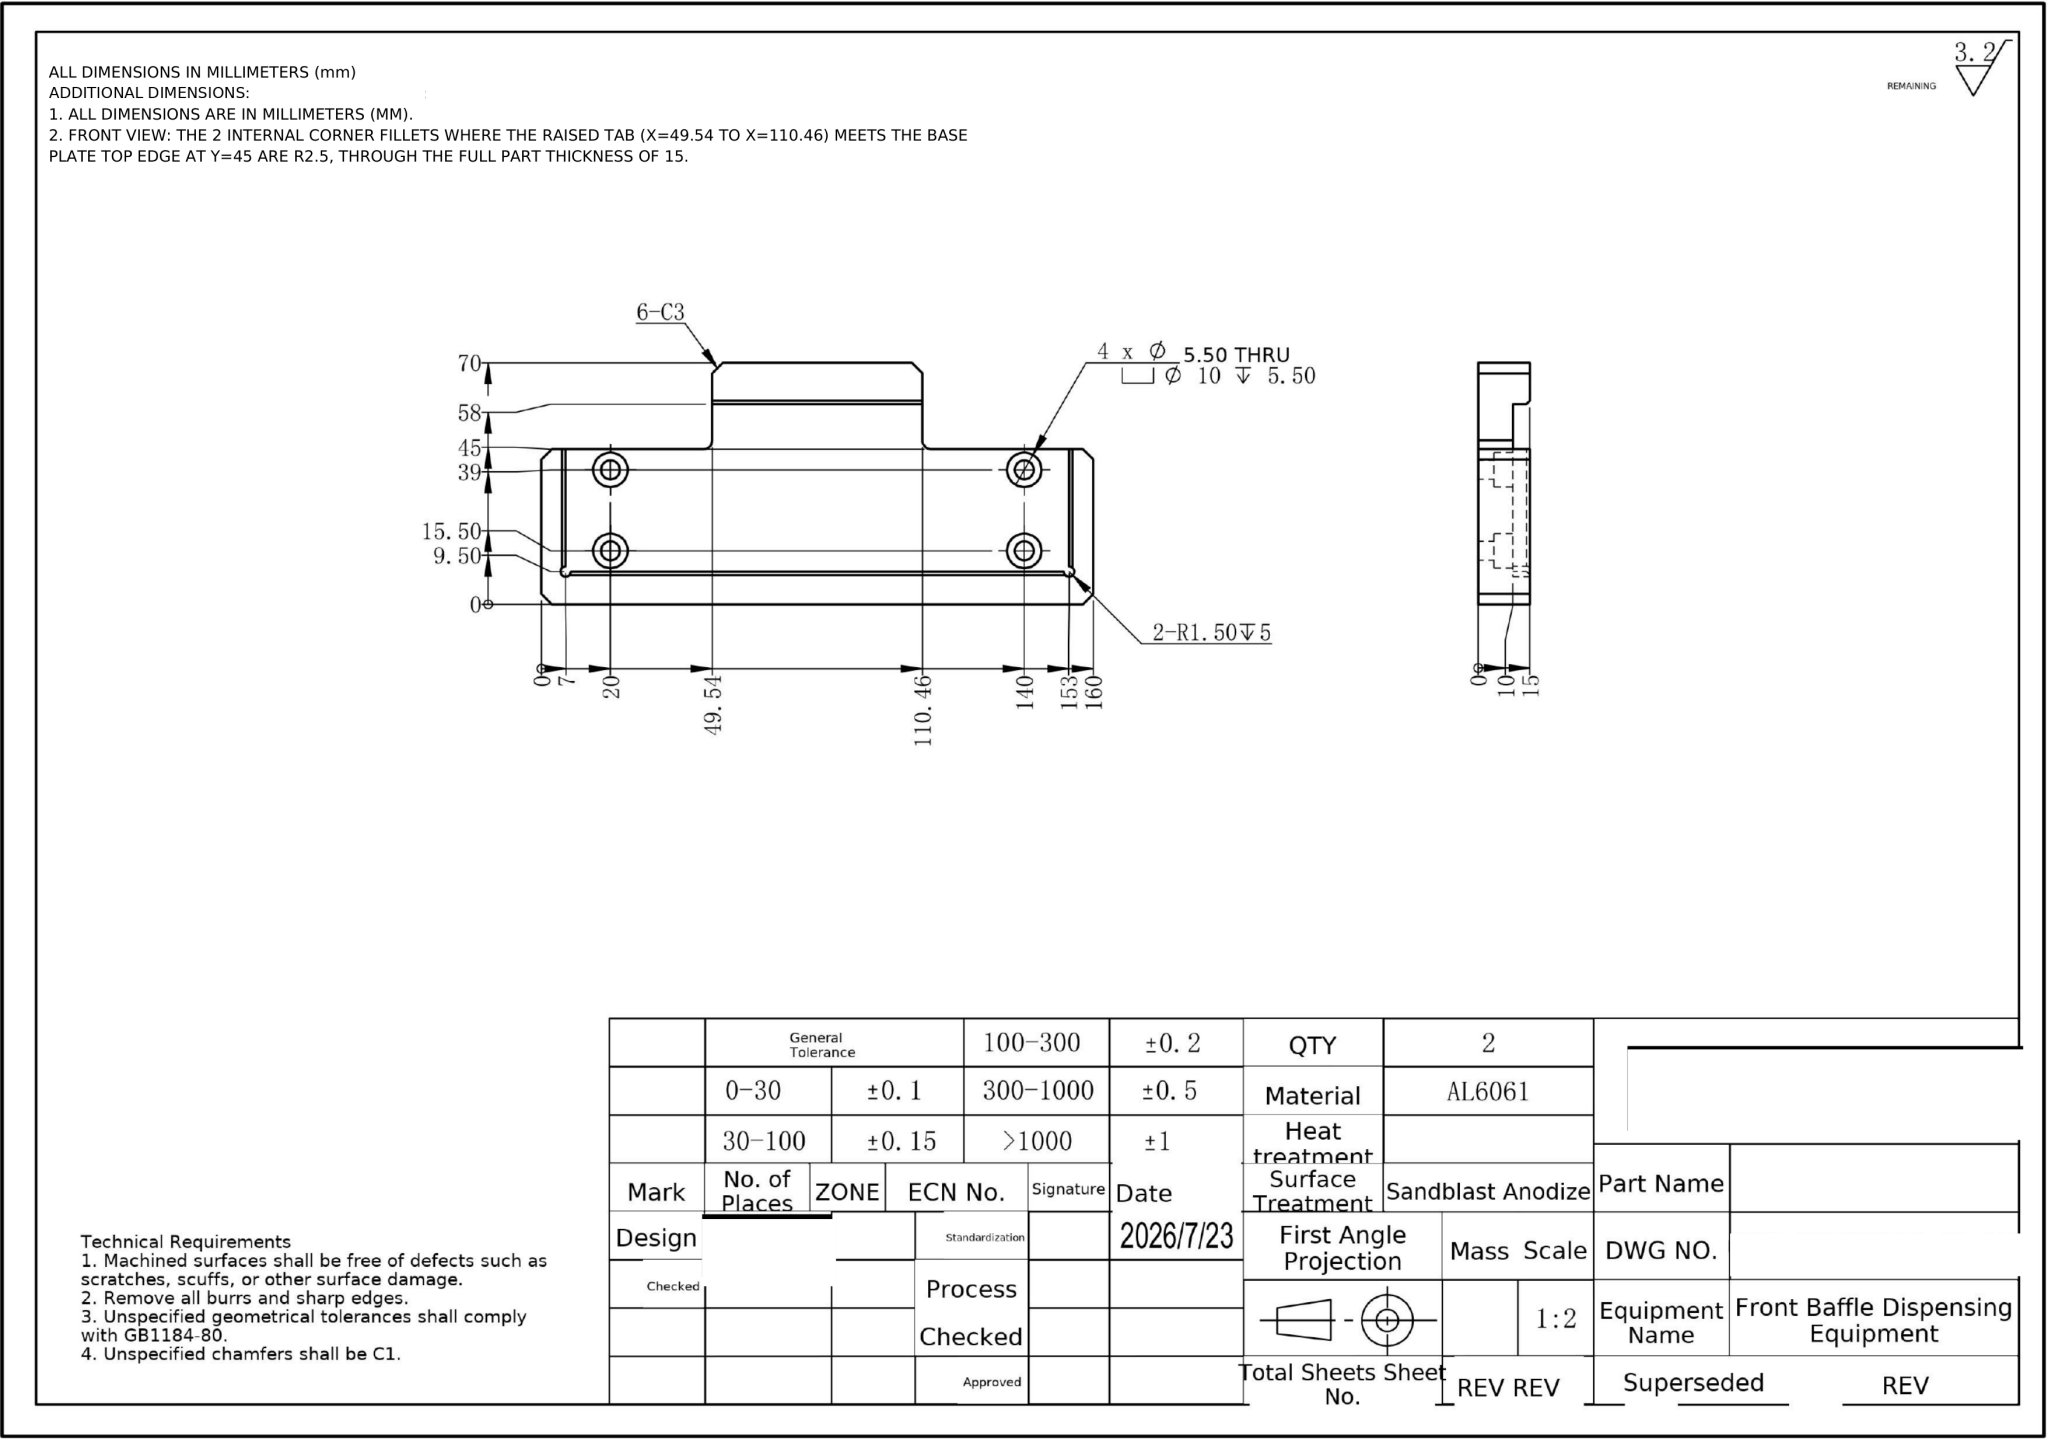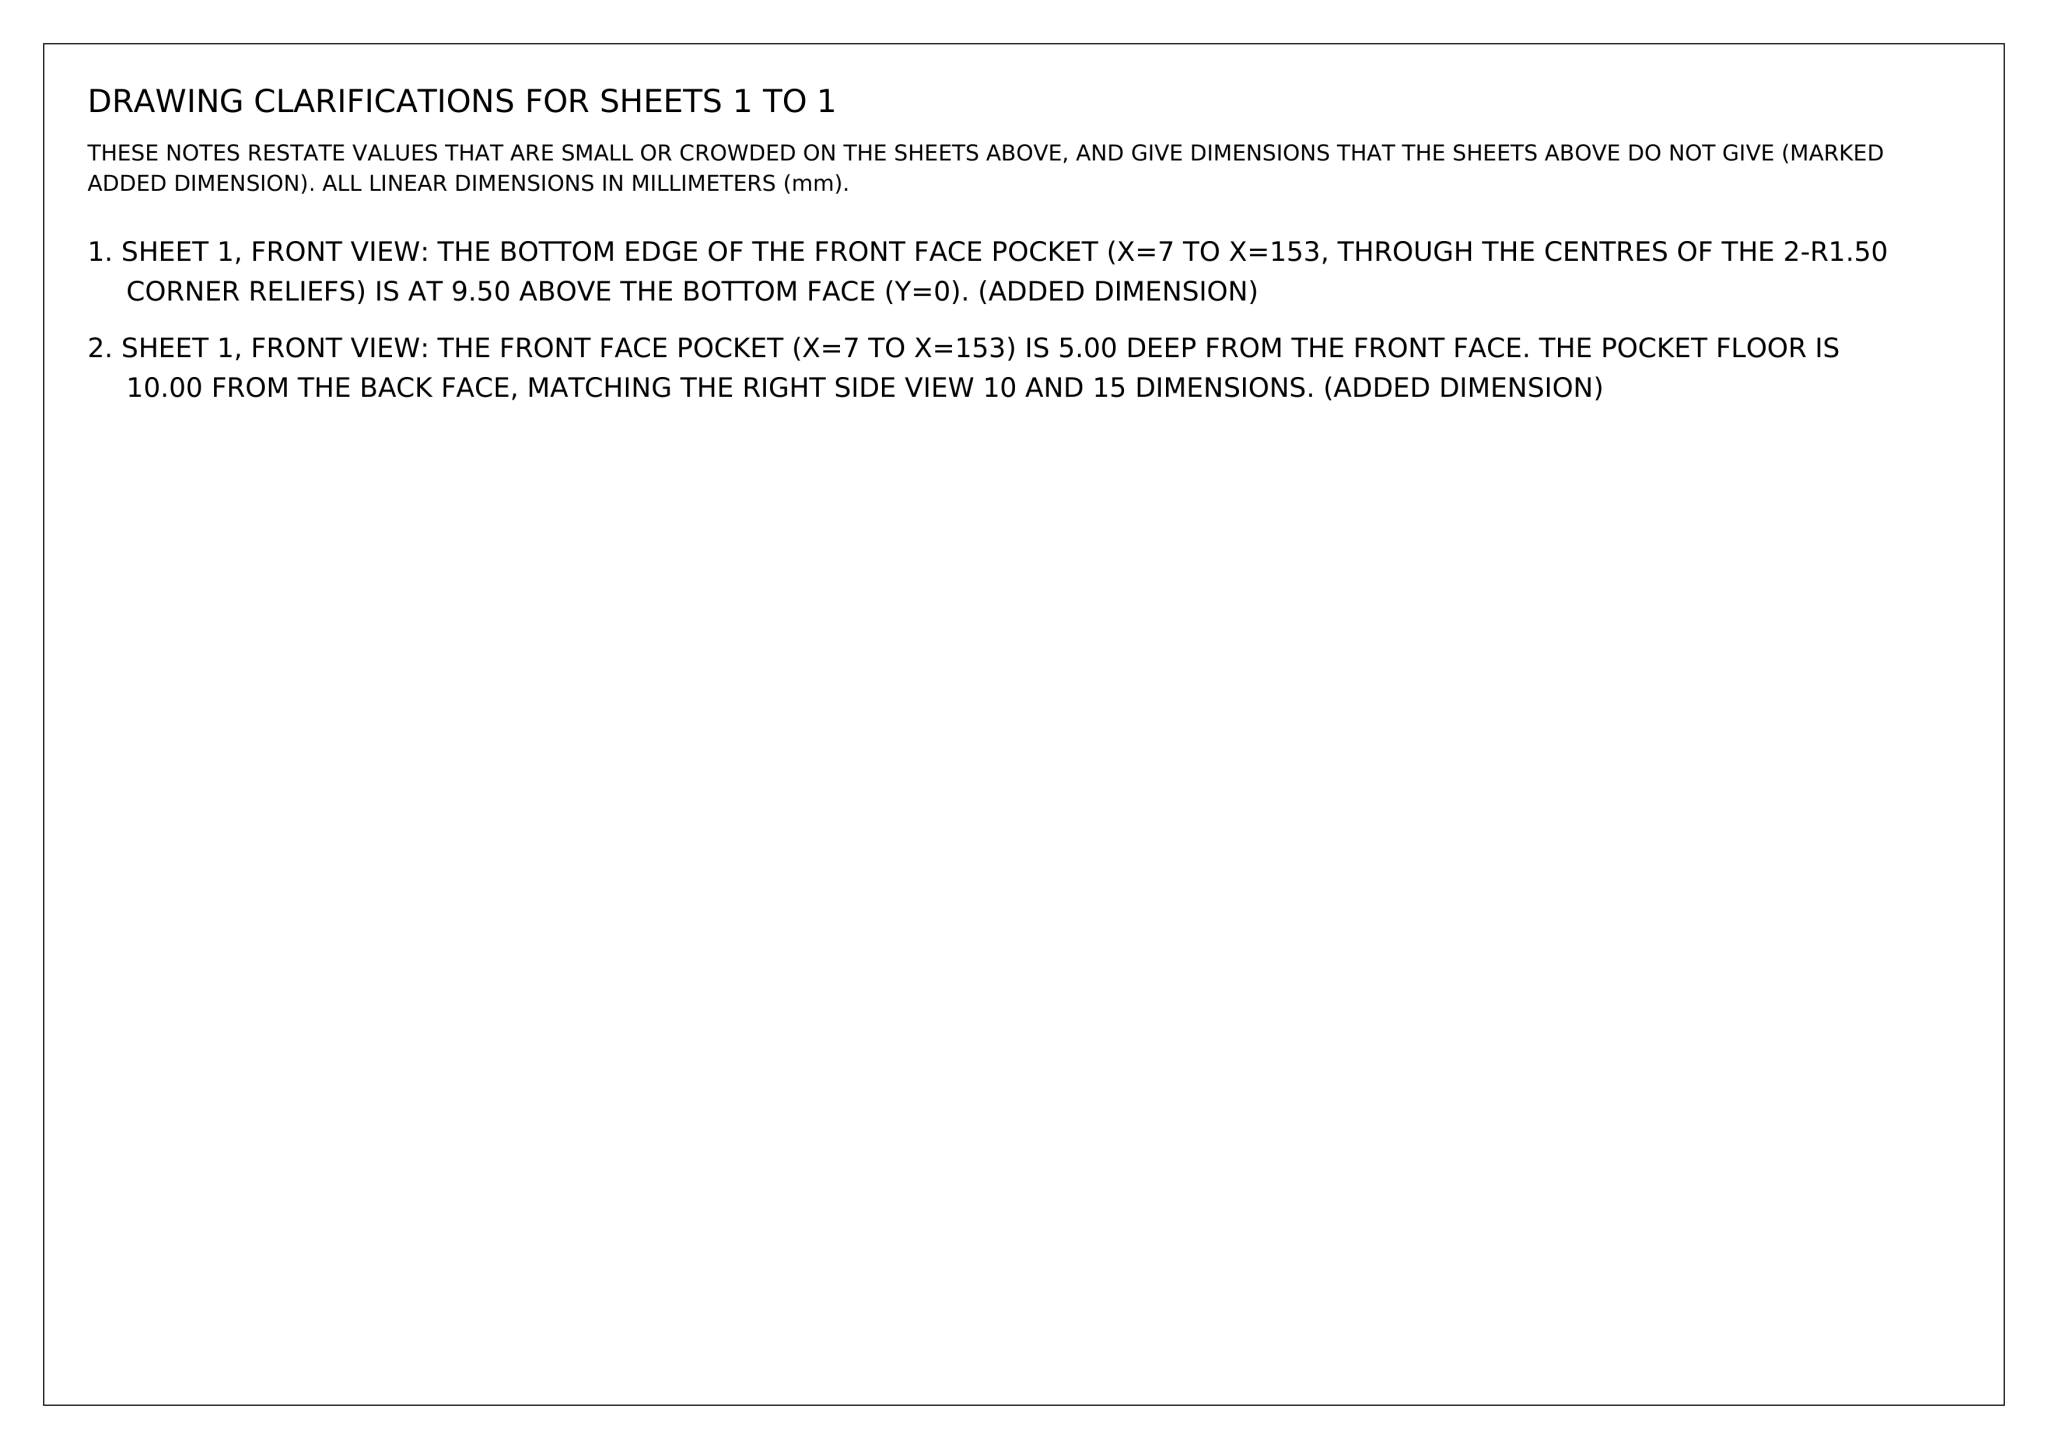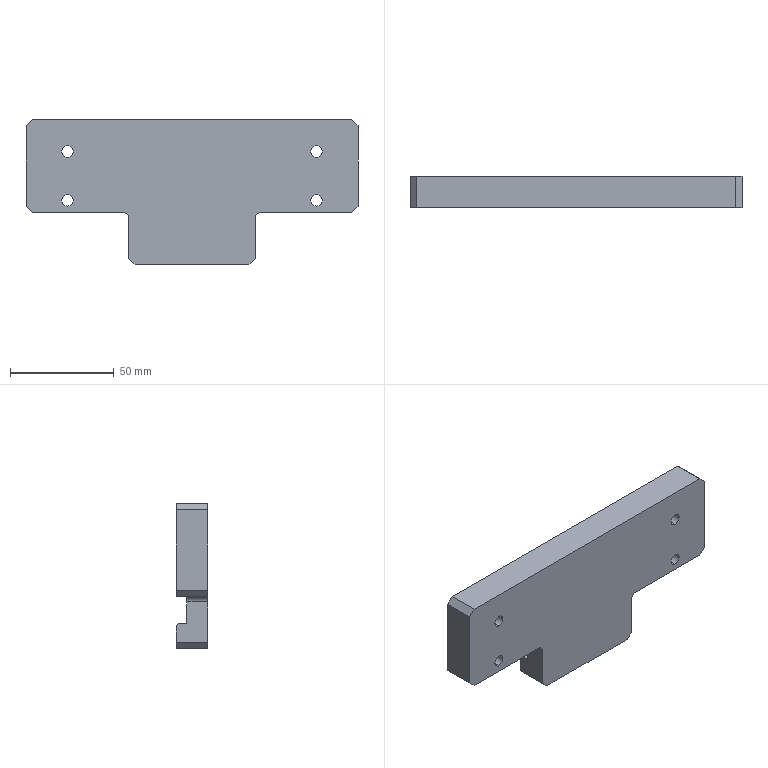Part | NX | mm | Angled Stepped Beam Bracket | 1 solid | 52 faces | box 160 x 15 x 70 mm | volume 98247 mm3 | plane 30 | cylinder 22 | commonest cylinder face diameters 10 x8 5.5 x8 3 x4 5 x2